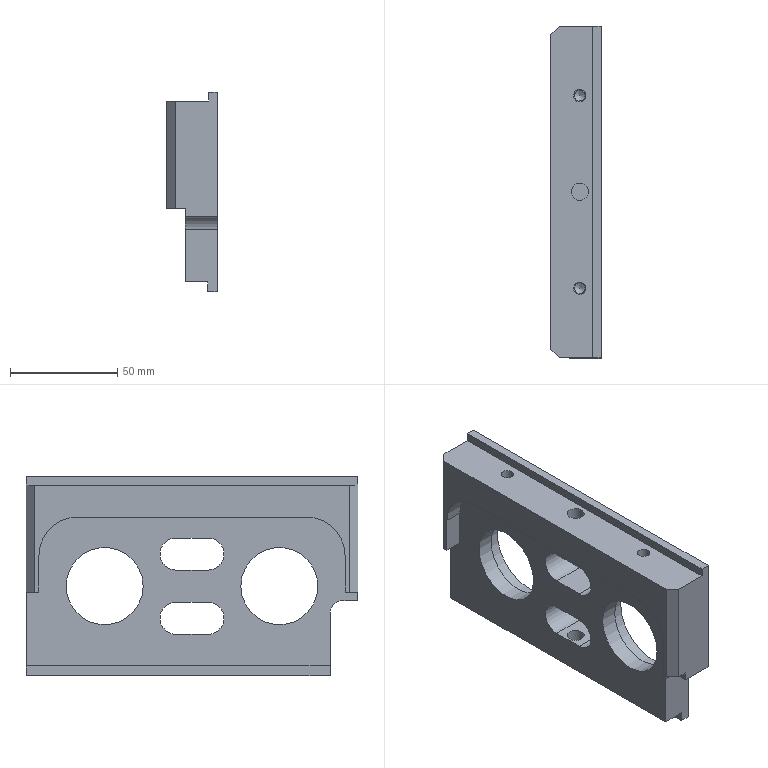Component | NX | LEFT_SIDE_PLATE | 1 solid | 55 faces | volume 168440 mm3 | plane 30 | cylinder 21 | cone 4 | commonest cylinder face diameters 15 x4 36 x4 5.795 x4 5 x4 42 x2 8 x2 12 x1